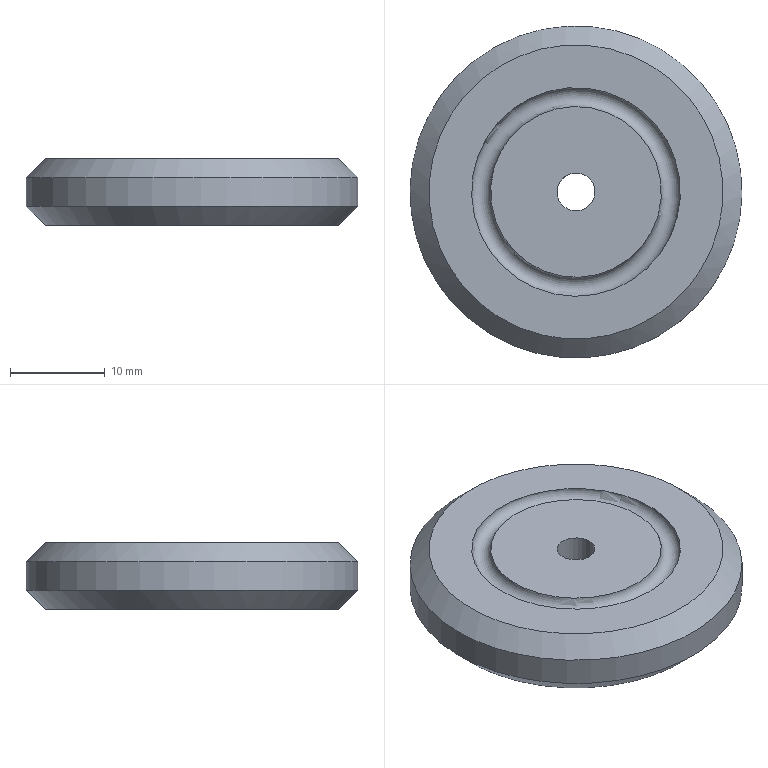Component | NX | SPRING_SEAT | 1 solid | 9 faces | box 35 x 35 x 7 mm | volume 6040 mm3 | cone 3 | plane 3 | cylinder 2 | torus 1 | commonest cylinder face diameters 4 x1 35 x1
STEP:
#1=CARTESIAN_POINT('',(0.,0.,0.));
#2=DIRECTION('',(0.,0.,1.));
#3=DIRECTION('',(1.,0.,0.));
#4=AXIS2_PLACEMENT_3D('',#1,#2,#3);
#5=CARTESIAN_POINT('',(-147.543,-1.847,125.));
#6=VERTEX_POINT('',#5);
#7=CARTESIAN_POINT('',(-146.777,0.,125.));
#8=DIRECTION('',(0.,0.,-1.));
#9=DIRECTION('',(-0.383,-0.9237,0.));
#10=AXIS2_PLACEMENT_3D('',#7,#8,#9);
#11=CIRCLE('',#10,2.);
#12=CARTESIAN_POINT('',(-146.777,0.,122.));
#13=DIRECTION('',(0.,0.,-1.));
#14=DIRECTION('',(-0.383,-0.9237,0.));
#15=AXIS2_PLACEMENT_3D('',#12,#13,#14);
#16=CYLINDRICAL_SURFACE('',#15,2.);
#17=CARTESIAN_POINT('',(0.,-3.));
#18=DIRECTION('',(1.,0.));
#19=VECTOR('',#18,1.);
#20=LINE('',#17,#19);
#21=(GEOMETRIC_REPRESENTATION_CONTEXT(2)PARAMETRIC_REPRESENTATION_CONTEXT()REPRESENTATION_CONTEXT('',''));
#22=DEFINITIONAL_REPRESENTATION('',(#20),#21);
#23=PCURVE('',#16,#22);
#24=CARTESIAN_POINT('',(-146.777,0.,125.));
#25=DIRECTION('',(0.,0.,-1.));
#26=DIRECTION('',(-0.383,-0.9237,0.));
#27=AXIS2_PLACEMENT_3D('',#24,#25,#26);
#28=CONICAL_SURFACE('',#27,2.,0.7854);
#29=CARTESIAN_POINT('',(0.,0.));
#30=DIRECTION('',(1.,0.));
#31=VECTOR('',#30,1.);
#32=LINE('',#29,#31);
#33=(GEOMETRIC_REPRESENTATION_CONTEXT(2)PARAMETRIC_REPRESENTATION_CONTEXT()REPRESENTATION_CONTEXT('',''));
#34=DEFINITIONAL_REPRESENTATION('',(#32),#33);
#35=PCURVE('',#28,#34);
#36=SURFACE_CURVE('',#11,(#23,#35),.PCURVE_S1.);
#37=EDGE_CURVE('',#6,#6,#36,.T.);
#38=ORIENTED_EDGE('',*,*,#37,.F.);
#39=CARTESIAN_POINT('',(-147.543,-1.847,129.));
#40=VERTEX_POINT('',#39);
#41=CARTESIAN_POINT('',(-147.543,-1.847,129.));
#42=CARTESIAN_POINT('',(-147.543,-1.847,125.));
#43=B_SPLINE_CURVE_WITH_KNOTS('',1,(#41,#42),.UNSPECIFIED.,.F.,.F.,(2,2),(-7.,-3.),.PIECEWISE_BEZIER_KNOTS.);
#44=CARTESIAN_POINT('',(0.,0.));
#45=DIRECTION('',(0.,1.));
#46=VECTOR('',#45,1.);
#47=LINE('',#44,#46);
#48=(GEOMETRIC_REPRESENTATION_CONTEXT(2)PARAMETRIC_REPRESENTATION_CONTEXT()REPRESENTATION_CONTEXT('',''));
#49=DEFINITIONAL_REPRESENTATION('',(#47),#48);
#50=PCURVE('',#16,#49);
#51=CARTESIAN_POINT('',(6.283,0.));
#52=DIRECTION('',(0.,1.));
#53=VECTOR('',#52,1.);
#54=LINE('',#51,#53);
#55=(GEOMETRIC_REPRESENTATION_CONTEXT(2)PARAMETRIC_REPRESENTATION_CONTEXT()REPRESENTATION_CONTEXT('',''));
#56=DEFINITIONAL_REPRESENTATION('',(#54),#55);
#57=PCURVE('',#16,#56);
#58=SEAM_CURVE('',#43,(#50,#57),.PCURVE_S1.);
#59=EDGE_CURVE('',#40,#6,#58,.T.);
#60=ORIENTED_EDGE('',*,*,#59,.F.);
#61=CARTESIAN_POINT('',(-146.777,0.,129.));
#62=DIRECTION('',(0.,0.,-1.));
#63=DIRECTION('',(-0.383,-0.9237,0.));
#64=AXIS2_PLACEMENT_3D('',#61,#62,#63);
#65=CIRCLE('',#64,2.);
#66=CARTESIAN_POINT('',(0.,-7.));
#67=DIRECTION('',(1.,0.));
#68=VECTOR('',#67,1.);
#69=LINE('',#66,#68);
#70=(GEOMETRIC_REPRESENTATION_CONTEXT(2)PARAMETRIC_REPRESENTATION_CONTEXT()REPRESENTATION_CONTEXT('',''));
#71=DEFINITIONAL_REPRESENTATION('',(#69),#70);
#72=PCURVE('',#16,#71);
#73=CARTESIAN_POINT('',(-155.091,3.447,129.));
#74=DIRECTION('',(0.,0.,1.));
#75=DIRECTION('',(0.383,0.9237,0.));
#76=AXIS2_PLACEMENT_3D('',#73,#74,#75);
#77=PLANE('',#76);
#78=CARTESIAN_POINT('',(-2.,-9.));
#79=CARTESIAN_POINT('',(-2.,-5.536));
#80=CARTESIAN_POINT('',(1.,-7.268));
#81=CARTESIAN_POINT('',(4.,-9.));
#82=CARTESIAN_POINT('',(1.,-10.732));
#83=CARTESIAN_POINT('',(-2.,-12.464));
#84=CARTESIAN_POINT('',(-2.,-9.));
#85=(BOUNDED_CURVE()B_SPLINE_CURVE(2,(#78,#79,#80,#81,#82,#83,#84),.UNSPECIFIED.,.T.,.F.)B_SPLINE_CURVE_WITH_KNOTS((1,2,2,2,2,1),(-2.094,0.,2.094,4.189,6.283,8.378),.UNSPECIFIED.)CURVE()GEOMETRIC_REPRESENTATION_ITEM()RATIONAL_B_SPLINE_CURVE((1.,0.5,1.,0.5,1.,0.5,1.))REPRESENTATION_ITEM(''));
#86=(GEOMETRIC_REPRESENTATION_CONTEXT(2)PARAMETRIC_REPRESENTATION_CONTEXT()REPRESENTATION_CONTEXT('',''));
#87=DEFINITIONAL_REPRESENTATION('',(#85),#86);
#88=PCURVE('',#77,#87);
#89=SURFACE_CURVE('',#65,(#72,#88),.PCURVE_S1.);
#90=EDGE_CURVE('',#40,#40,#89,.T.);
#91=ORIENTED_EDGE('',*,*,#90,.T.);
#92=ORIENTED_EDGE('',*,*,#59,.T.);
#93=EDGE_LOOP('',(#38,#60,#91,#92));
#94=FACE_BOUND('',#93,.F.);
#95=ADVANCED_FACE('',(#94),#16,.F.);
#96=CARTESIAN_POINT('',(-148.693,-4.619,122.));
#97=VERTEX_POINT('',#96);
#98=CARTESIAN_POINT('',(-146.777,0.,122.));
#99=DIRECTION('',(0.,0.,-1.));
#100=DIRECTION('',(-0.383,-0.9237,0.));
#101=AXIS2_PLACEMENT_3D('',#98,#99,#100);
#102=CIRCLE('',#101,5.);
#103=CARTESIAN_POINT('',(0.,3.));
#104=DIRECTION('',(1.,0.));
#105=VECTOR('',#104,1.);
#106=LINE('',#103,#105);
#107=(GEOMETRIC_REPRESENTATION_CONTEXT(2)PARAMETRIC_REPRESENTATION_CONTEXT()REPRESENTATION_CONTEXT('',''));
#108=DEFINITIONAL_REPRESENTATION('',(#106),#107);
#109=PCURVE('',#28,#108);
#110=CARTESIAN_POINT('',(-151.396,1.915,122.));
#111=DIRECTION('',(0.,0.,-1.));
#112=DIRECTION('',(-0.383,-0.9237,0.));
#113=AXIS2_PLACEMENT_3D('',#110,#111,#112);
#114=PLANE('',#113);
#115=CARTESIAN_POINT('',(-0.,-5.));
#116=DIRECTION('',(1.,-0.));
#117=AXIS2_PLACEMENT_2D('',#115,#116);
#118=CIRCLE('',#117,5.);
#119=(GEOMETRIC_REPRESENTATION_CONTEXT(2)PARAMETRIC_REPRESENTATION_CONTEXT()REPRESENTATION_CONTEXT('',''));
#120=DEFINITIONAL_REPRESENTATION('',(#118),#119);
#121=PCURVE('',#114,#120);
#122=SURFACE_CURVE('',#102,(#109,#121),.PCURVE_S1.);
#123=EDGE_CURVE('',#97,#97,#122,.T.);
#124=ORIENTED_EDGE('',*,*,#123,.F.);
#125=CARTESIAN_POINT('',(-147.543,-1.847,125.));
#126=CARTESIAN_POINT('',(-148.693,-4.619,122.));
#127=B_SPLINE_CURVE_WITH_KNOTS('',1,(#125,#126),.UNSPECIFIED.,.F.,.F.,(2,2),(0.,4.243),.PIECEWISE_BEZIER_KNOTS.);
#128=CARTESIAN_POINT('',(0.,0.));
#129=DIRECTION('',(0.,1.));
#130=VECTOR('',#129,1.);
#131=LINE('',#128,#130);
#132=(GEOMETRIC_REPRESENTATION_CONTEXT(2)PARAMETRIC_REPRESENTATION_CONTEXT()REPRESENTATION_CONTEXT('',''));
#133=DEFINITIONAL_REPRESENTATION('',(#131),#132);
#134=PCURVE('',#28,#133);
#135=CARTESIAN_POINT('',(6.283,0.));
#136=DIRECTION('',(0.,1.));
#137=VECTOR('',#136,1.);
#138=LINE('',#135,#137);
#139=(GEOMETRIC_REPRESENTATION_CONTEXT(2)PARAMETRIC_REPRESENTATION_CONTEXT()REPRESENTATION_CONTEXT('',''));
#140=DEFINITIONAL_REPRESENTATION('',(#138),#139);
#141=PCURVE('',#28,#140);
#142=SEAM_CURVE('',#127,(#134,#141),.PCURVE_S1.);
#143=EDGE_CURVE('',#6,#97,#142,.T.);
#144=ORIENTED_EDGE('',*,*,#143,.F.);
#145=ORIENTED_EDGE('',*,*,#37,.T.);
#146=ORIENTED_EDGE('',*,*,#143,.T.);
#147=EDGE_LOOP('',(#124,#144,#145,#146));
#148=FACE_BOUND('',#147,.F.);
#149=ADVANCED_FACE('',(#148),#28,.F.);
#150=CARTESIAN_POINT('',(-152.715,-14.318,122.));
#151=VERTEX_POINT('',#150);
#152=CARTESIAN_POINT('',(-146.777,0.,122.));
#153=DIRECTION('',(0.,0.,-1.));
#154=DIRECTION('',(-0.383,-0.9237,0.));
#155=AXIS2_PLACEMENT_3D('',#152,#153,#154);
#156=CIRCLE('',#155,15.5);
#157=CARTESIAN_POINT('',(-0.,-5.));
#158=DIRECTION('',(1.,0.));
#159=AXIS2_PLACEMENT_2D('',#157,#158);
#160=CIRCLE('',#159,15.5);
#161=(GEOMETRIC_REPRESENTATION_CONTEXT(2)PARAMETRIC_REPRESENTATION_CONTEXT()REPRESENTATION_CONTEXT('',''));
#162=DEFINITIONAL_REPRESENTATION('',(#160),#161);
#163=PCURVE('',#114,#162);
#164=CARTESIAN_POINT('',(-146.777,0.,122.));
#165=DIRECTION('',(0.,0.,1.));
#166=DIRECTION('',(0.383,0.9237,0.));
#167=AXIS2_PLACEMENT_3D('',#164,#165,#166);
#168=CONICAL_SURFACE('',#167,15.5,0.7854);
#169=CARTESIAN_POINT('',(9.425,0.));
#170=DIRECTION('',(-1.,0.));
#171=VECTOR('',#170,1.);
#172=LINE('',#169,#171);
#173=(GEOMETRIC_REPRESENTATION_CONTEXT(2)PARAMETRIC_REPRESENTATION_CONTEXT()REPRESENTATION_CONTEXT('',''));
#174=DEFINITIONAL_REPRESENTATION('',(#172),#173);
#175=PCURVE('',#168,#174);
#176=SURFACE_CURVE('',#156,(#163,#175),.PCURVE_S1.);
#177=EDGE_CURVE('',#151,#151,#176,.T.);
#178=ORIENTED_EDGE('',*,*,#177,.T.);
#179=EDGE_LOOP('',(#178));
#180=FACE_BOUND('',#179,.T.);
#181=ORIENTED_EDGE('',*,*,#123,.F.);
#182=EDGE_LOOP('',(#181));
#183=FACE_BOUND('',#182,.T.);
#184=ADVANCED_FACE('',(#180,#183),#114,.T.);
#185=CARTESIAN_POINT('',(-153.481,-16.165,124.));
#186=VERTEX_POINT('',#185);
#187=CARTESIAN_POINT('',(-146.777,0.,124.));
#188=DIRECTION('',(0.,0.,-1.));
#189=DIRECTION('',(-0.383,-0.9237,0.));
#190=AXIS2_PLACEMENT_3D('',#187,#188,#189);
#191=CIRCLE('',#190,17.5);
#192=CARTESIAN_POINT('',(9.425,2.));
#193=DIRECTION('',(-1.,0.));
#194=VECTOR('',#193,1.);
#195=LINE('',#192,#194);
#196=(GEOMETRIC_REPRESENTATION_CONTEXT(2)PARAMETRIC_REPRESENTATION_CONTEXT()REPRESENTATION_CONTEXT('',''));
#197=DEFINITIONAL_REPRESENTATION('',(#195),#196);
#198=PCURVE('',#168,#197);
#199=CARTESIAN_POINT('',(-146.777,0.,122.));
#200=DIRECTION('',(0.,0.,-1.));
#201=DIRECTION('',(-0.383,-0.9237,0.));
#202=AXIS2_PLACEMENT_3D('',#199,#200,#201);
#203=CYLINDRICAL_SURFACE('',#202,17.5);
#204=CARTESIAN_POINT('',(0.,-2.));
#205=DIRECTION('',(1.,0.));
#206=VECTOR('',#205,1.);
#207=LINE('',#204,#206);
#208=(GEOMETRIC_REPRESENTATION_CONTEXT(2)PARAMETRIC_REPRESENTATION_CONTEXT()REPRESENTATION_CONTEXT('',''));
#209=DEFINITIONAL_REPRESENTATION('',(#207),#208);
#210=PCURVE('',#203,#209);
#211=SURFACE_CURVE('',#191,(#198,#210),.PCURVE_S1.);
#212=EDGE_CURVE('',#186,#186,#211,.T.);
#213=ORIENTED_EDGE('',*,*,#212,.T.);
#214=CARTESIAN_POINT('',(-152.715,-14.318,122.));
#215=CARTESIAN_POINT('',(-153.481,-16.165,124.));
#216=B_SPLINE_CURVE_WITH_KNOTS('',1,(#214,#215),.UNSPECIFIED.,.F.,.F.,(2,2),(0.,2.828),.PIECEWISE_BEZIER_KNOTS.);
#217=CARTESIAN_POINT('',(3.142,0.));
#218=DIRECTION('',(0.,1.));
#219=VECTOR('',#218,1.);
#220=LINE('',#217,#219);
#221=(GEOMETRIC_REPRESENTATION_CONTEXT(2)PARAMETRIC_REPRESENTATION_CONTEXT()REPRESENTATION_CONTEXT('',''));
#222=DEFINITIONAL_REPRESENTATION('',(#220),#221);
#223=PCURVE('',#168,#222);
#224=CARTESIAN_POINT('',(9.425,0.));
#225=DIRECTION('',(0.,1.));
#226=VECTOR('',#225,1.);
#227=LINE('',#224,#226);
#228=(GEOMETRIC_REPRESENTATION_CONTEXT(2)PARAMETRIC_REPRESENTATION_CONTEXT()REPRESENTATION_CONTEXT('',''));
#229=DEFINITIONAL_REPRESENTATION('',(#227),#228);
#230=PCURVE('',#168,#229);
#231=SEAM_CURVE('',#216,(#223,#230),.PCURVE_S1.);
#232=EDGE_CURVE('',#151,#186,#231,.T.);
#233=ORIENTED_EDGE('',*,*,#232,.F.);
#234=ORIENTED_EDGE('',*,*,#177,.F.);
#235=ORIENTED_EDGE('',*,*,#232,.T.);
#236=EDGE_LOOP('',(#213,#233,#234,#235));
#237=FACE_BOUND('',#236,.T.);
#238=ADVANCED_FACE('',(#237),#168,.T.);
#239=CARTESIAN_POINT('',(-153.481,-16.165,127.));
#240=VERTEX_POINT('',#239);
#241=CARTESIAN_POINT('',(-146.777,0.,127.));
#242=DIRECTION('',(0.,0.,-1.));
#243=DIRECTION('',(-0.383,-0.9237,0.));
#244=AXIS2_PLACEMENT_3D('',#241,#242,#243);
#245=CIRCLE('',#244,17.5);
#246=CARTESIAN_POINT('',(0.,-5.));
#247=DIRECTION('',(1.,0.));
#248=VECTOR('',#247,1.);
#249=LINE('',#246,#248);
#250=(GEOMETRIC_REPRESENTATION_CONTEXT(2)PARAMETRIC_REPRESENTATION_CONTEXT()REPRESENTATION_CONTEXT('',''));
#251=DEFINITIONAL_REPRESENTATION('',(#249),#250);
#252=PCURVE('',#203,#251);
#253=CARTESIAN_POINT('',(-146.777,0.,127.));
#254=DIRECTION('',(0.,0.,-1.));
#255=DIRECTION('',(-0.383,-0.9237,0.));
#256=AXIS2_PLACEMENT_3D('',#253,#254,#255);
#257=CONICAL_SURFACE('',#256,17.5,0.7854);
#258=CARTESIAN_POINT('',(0.,0.));
#259=DIRECTION('',(1.,0.));
#260=VECTOR('',#259,1.);
#261=LINE('',#258,#260);
#262=(GEOMETRIC_REPRESENTATION_CONTEXT(2)PARAMETRIC_REPRESENTATION_CONTEXT()REPRESENTATION_CONTEXT('',''));
#263=DEFINITIONAL_REPRESENTATION('',(#261),#262);
#264=PCURVE('',#257,#263);
#265=SURFACE_CURVE('',#245,(#252,#264),.PCURVE_S1.);
#266=EDGE_CURVE('',#240,#240,#265,.T.);
#267=ORIENTED_EDGE('',*,*,#266,.T.);
#268=CARTESIAN_POINT('',(-153.481,-16.165,127.));
#269=CARTESIAN_POINT('',(-153.481,-16.165,124.));
#270=B_SPLINE_CURVE_WITH_KNOTS('',1,(#268,#269),.UNSPECIFIED.,.F.,.F.,(2,2),(-5.,-2.),.PIECEWISE_BEZIER_KNOTS.);
#271=CARTESIAN_POINT('',(6.283,0.));
#272=DIRECTION('',(0.,1.));
#273=VECTOR('',#272,1.);
#274=LINE('',#271,#273);
#275=(GEOMETRIC_REPRESENTATION_CONTEXT(2)PARAMETRIC_REPRESENTATION_CONTEXT()REPRESENTATION_CONTEXT('',''));
#276=DEFINITIONAL_REPRESENTATION('',(#274),#275);
#277=PCURVE('',#203,#276);
#278=CARTESIAN_POINT('',(0.,0.));
#279=DIRECTION('',(0.,1.));
#280=VECTOR('',#279,1.);
#281=LINE('',#278,#280);
#282=(GEOMETRIC_REPRESENTATION_CONTEXT(2)PARAMETRIC_REPRESENTATION_CONTEXT()REPRESENTATION_CONTEXT('',''));
#283=DEFINITIONAL_REPRESENTATION('',(#281),#282);
#284=PCURVE('',#203,#283);
#285=SEAM_CURVE('',#270,(#277,#284),.PCURVE_S1.);
#286=EDGE_CURVE('',#240,#186,#285,.T.);
#287=ORIENTED_EDGE('',*,*,#286,.T.);
#288=ORIENTED_EDGE('',*,*,#212,.F.);
#289=ORIENTED_EDGE('',*,*,#286,.F.);
#290=EDGE_LOOP('',(#267,#287,#288,#289));
#291=FACE_BOUND('',#290,.T.);
#292=ADVANCED_FACE('',(#291),#203,.T.);
#293=CARTESIAN_POINT('',(-152.715,-14.318,129.));
#294=VERTEX_POINT('',#293);
#295=CARTESIAN_POINT('',(-146.777,0.,129.));
#296=DIRECTION('',(0.,0.,-1.));
#297=DIRECTION('',(-0.383,-0.9237,0.));
#298=AXIS2_PLACEMENT_3D('',#295,#296,#297);
#299=CIRCLE('',#298,15.5);
#300=CARTESIAN_POINT('',(0.,-2.));
#301=DIRECTION('',(1.,0.));
#302=VECTOR('',#301,1.);
#303=LINE('',#300,#302);
#304=(GEOMETRIC_REPRESENTATION_CONTEXT(2)PARAMETRIC_REPRESENTATION_CONTEXT()REPRESENTATION_CONTEXT('',''));
#305=DEFINITIONAL_REPRESENTATION('',(#303),#304);
#306=PCURVE('',#257,#305);
#307=CARTESIAN_POINT('',(-161.095,5.937,129.));
#308=DIRECTION('',(0.,0.,1.));
#309=DIRECTION('',(0.383,0.9237,0.));
#310=AXIS2_PLACEMENT_3D('',#307,#308,#309);
#311=PLANE('',#310);
#312=CARTESIAN_POINT('',(-15.5,-15.5));
#313=CARTESIAN_POINT('',(-15.5,11.347));
#314=CARTESIAN_POINT('',(7.75,-2.077));
#315=CARTESIAN_POINT('',(31.,-15.5));
#316=CARTESIAN_POINT('',(7.75,-28.923));
#317=CARTESIAN_POINT('',(-15.5,-42.347));
#318=CARTESIAN_POINT('',(-15.5,-15.5));
#319=(BOUNDED_CURVE()B_SPLINE_CURVE(2,(#312,#313,#314,#315,#316,#317,#318),.UNSPECIFIED.,.T.,.F.)B_SPLINE_CURVE_WITH_KNOTS((1,2,2,2,2,1),(-2.094,0.,2.094,4.189,6.283,8.378),.UNSPECIFIED.)CURVE()GEOMETRIC_REPRESENTATION_ITEM()RATIONAL_B_SPLINE_CURVE((1.,0.5,1.,0.5,1.,0.5,1.))REPRESENTATION_ITEM(''));
#320=(GEOMETRIC_REPRESENTATION_CONTEXT(2)PARAMETRIC_REPRESENTATION_CONTEXT()REPRESENTATION_CONTEXT('',''));
#321=DEFINITIONAL_REPRESENTATION('',(#319),#320);
#322=PCURVE('',#311,#321);
#323=SURFACE_CURVE('',#299,(#306,#322),.PCURVE_S1.);
#324=EDGE_CURVE('',#294,#294,#323,.T.);
#325=ORIENTED_EDGE('',*,*,#324,.T.);
#326=CARTESIAN_POINT('',(-152.715,-14.318,129.));
#327=CARTESIAN_POINT('',(-153.481,-16.165,127.));
#328=B_SPLINE_CURVE_WITH_KNOTS('',1,(#326,#327),.UNSPECIFIED.,.F.,.F.,(2,2),(-2.828,0.),.PIECEWISE_BEZIER_KNOTS.);
#329=CARTESIAN_POINT('',(6.283,0.));
#330=DIRECTION('',(0.,1.));
#331=VECTOR('',#330,1.);
#332=LINE('',#329,#331);
#333=(GEOMETRIC_REPRESENTATION_CONTEXT(2)PARAMETRIC_REPRESENTATION_CONTEXT()REPRESENTATION_CONTEXT('',''));
#334=DEFINITIONAL_REPRESENTATION('',(#332),#333);
#335=PCURVE('',#257,#334);
#336=CARTESIAN_POINT('',(0.,0.));
#337=DIRECTION('',(0.,1.));
#338=VECTOR('',#337,1.);
#339=LINE('',#336,#338);
#340=(GEOMETRIC_REPRESENTATION_CONTEXT(2)PARAMETRIC_REPRESENTATION_CONTEXT()REPRESENTATION_CONTEXT('',''));
#341=DEFINITIONAL_REPRESENTATION('',(#339),#340);
#342=PCURVE('',#257,#341);
#343=SEAM_CURVE('',#328,(#335,#342),.PCURVE_S1.);
#344=EDGE_CURVE('',#294,#240,#343,.T.);
#345=ORIENTED_EDGE('',*,*,#344,.T.);
#346=ORIENTED_EDGE('',*,*,#266,.F.);
#347=ORIENTED_EDGE('',*,*,#344,.F.);
#348=EDGE_LOOP('',(#325,#345,#346,#347));
#349=FACE_BOUND('',#348,.T.);
#350=ADVANCED_FACE('',(#349),#257,.T.);
#351=CARTESIAN_POINT('',(-150.991,-10.161,129.));
#352=VERTEX_POINT('',#351);
#353=CARTESIAN_POINT('',(-146.777,0.,129.));
#354=DIRECTION('',(0.,0.,-1.));
#355=DIRECTION('',(-0.383,-0.9237,0.));
#356=AXIS2_PLACEMENT_3D('',#353,#354,#355);
#357=CIRCLE('',#356,11.);
#358=CARTESIAN_POINT('',(-11.,-15.5));
#359=CARTESIAN_POINT('',(-11.,3.553));
#360=CARTESIAN_POINT('',(5.5,-5.974));
#361=CARTESIAN_POINT('',(22.,-15.5));
#362=CARTESIAN_POINT('',(5.5,-25.026));
#363=CARTESIAN_POINT('',(-11.,-34.553));
#364=CARTESIAN_POINT('',(-11.,-15.5));
#365=(BOUNDED_CURVE()B_SPLINE_CURVE(2,(#358,#359,#360,#361,#362,#363,#364),.UNSPECIFIED.,.T.,.F.)B_SPLINE_CURVE_WITH_KNOTS((1,2,2,2,2,1),(-2.094,0.,2.094,4.189,6.283,8.378),.UNSPECIFIED.)CURVE()GEOMETRIC_REPRESENTATION_ITEM()RATIONAL_B_SPLINE_CURVE((1.,0.5,1.,0.5,1.,0.5,1.))REPRESENTATION_ITEM(''));
#366=(GEOMETRIC_REPRESENTATION_CONTEXT(2)PARAMETRIC_REPRESENTATION_CONTEXT()REPRESENTATION_CONTEXT('',''));
#367=DEFINITIONAL_REPRESENTATION('',(#365),#366);
#368=PCURVE('',#311,#367);
#369=CARTESIAN_POINT('',(-146.777,0.,129.));
#370=DIRECTION('',(0.,0.,-1.));
#371=DIRECTION('',(-0.383,-0.9237,0.));
#372=AXIS2_PLACEMENT_3D('',#369,#370,#371);
#373=TOROIDAL_SURFACE('',#372,10.,1.);
#374=CARTESIAN_POINT('',(0.,6.283));
#375=DIRECTION('',(1.,0.));
#376=VECTOR('',#375,1.);
#377=LINE('',#374,#376);
#378=(GEOMETRIC_REPRESENTATION_CONTEXT(2)PARAMETRIC_REPRESENTATION_CONTEXT()REPRESENTATION_CONTEXT('',''));
#379=DEFINITIONAL_REPRESENTATION('',(#377),#378);
#380=PCURVE('',#373,#379);
#381=SURFACE_CURVE('',#357,(#368,#380),.PCURVE_S1.);
#382=EDGE_CURVE('',#352,#352,#381,.T.);
#383=ORIENTED_EDGE('',*,*,#382,.T.);
#384=EDGE_LOOP('',(#383));
#385=FACE_BOUND('',#384,.T.);
#386=ORIENTED_EDGE('',*,*,#324,.F.);
#387=EDGE_LOOP('',(#386));
#388=FACE_BOUND('',#387,.T.);
#389=ADVANCED_FACE('',(#385,#388),#311,.T.);
#390=CARTESIAN_POINT('',(-150.225,-8.314,129.));
#391=VERTEX_POINT('',#390);
#392=CARTESIAN_POINT('',(-146.777,0.,129.));
#393=DIRECTION('',(0.,0.,-1.));
#394=DIRECTION('',(-0.383,-0.9237,0.));
#395=AXIS2_PLACEMENT_3D('',#392,#393,#394);
#396=CIRCLE('',#395,9.);
#397=CARTESIAN_POINT('',(0.,9.425));
#398=DIRECTION('',(1.,0.));
#399=VECTOR('',#398,1.);
#400=LINE('',#397,#399);
#401=(GEOMETRIC_REPRESENTATION_CONTEXT(2)PARAMETRIC_REPRESENTATION_CONTEXT()REPRESENTATION_CONTEXT('',''));
#402=DEFINITIONAL_REPRESENTATION('',(#400),#401);
#403=PCURVE('',#373,#402);
#404=CARTESIAN_POINT('',(-9.,-9.));
#405=CARTESIAN_POINT('',(-9.,6.588));
#406=CARTESIAN_POINT('',(4.5,-1.206));
#407=CARTESIAN_POINT('',(18.,-9.));
#408=CARTESIAN_POINT('',(4.5,-16.794));
#409=CARTESIAN_POINT('',(-9.,-24.588));
#410=CARTESIAN_POINT('',(-9.,-9.));
#411=(BOUNDED_CURVE()B_SPLINE_CURVE(2,(#404,#405,#406,#407,#408,#409,#410),.UNSPECIFIED.,.T.,.F.)B_SPLINE_CURVE_WITH_KNOTS((1,2,2,2,2,1),(-2.094,0.,2.094,4.189,6.283,8.378),.UNSPECIFIED.)CURVE()GEOMETRIC_REPRESENTATION_ITEM()RATIONAL_B_SPLINE_CURVE((1.,0.5,1.,0.5,1.,0.5,1.))REPRESENTATION_ITEM(''));
#412=(GEOMETRIC_REPRESENTATION_CONTEXT(2)PARAMETRIC_REPRESENTATION_CONTEXT()REPRESENTATION_CONTEXT('',''));
#413=DEFINITIONAL_REPRESENTATION('',(#411),#412);
#414=PCURVE('',#77,#413);
#415=SURFACE_CURVE('',#396,(#403,#414),.PCURVE_S1.);
#416=EDGE_CURVE('',#391,#391,#415,.T.);
#417=ORIENTED_EDGE('',*,*,#416,.F.);
#418=CARTESIAN_POINT('',(-150.991,-10.161,129.));
#419=CARTESIAN_POINT('',(-150.991,-10.161,128.607));
#420=CARTESIAN_POINT('',(-150.923,-9.998,128.215));
#421=CARTESIAN_POINT('',(-150.788,-9.673,127.914));
#422=CARTESIAN_POINT('',(-150.608,-9.237,127.798));
#423=CARTESIAN_POINT('',(-150.427,-8.802,127.914));
#424=CARTESIAN_POINT('',(-150.292,-8.476,128.215));
#425=CARTESIAN_POINT('',(-150.225,-8.314,128.607));
#426=CARTESIAN_POINT('',(-150.225,-8.314,129.));
#427=B_SPLINE_CURVE_WITH_KNOTS('',8,(#418,#419,#420,#421,#422,#423,#424,#425,#426),.UNSPECIFIED.,.F.,.F.,(9,9),(0.,3.142),.PIECEWISE_BEZIER_KNOTS.);
#428=CARTESIAN_POINT('',(0.,6.283));
#429=DIRECTION('',(0.,1.));
#430=VECTOR('',#429,1.);
#431=LINE('',#428,#430);
#432=(GEOMETRIC_REPRESENTATION_CONTEXT(2)PARAMETRIC_REPRESENTATION_CONTEXT()REPRESENTATION_CONTEXT('',''));
#433=DEFINITIONAL_REPRESENTATION('',(#431),#432);
#434=PCURVE('',#373,#433);
#435=CARTESIAN_POINT('',(6.283,6.283));
#436=DIRECTION('',(0.,1.));
#437=VECTOR('',#436,1.);
#438=LINE('',#435,#437);
#439=(GEOMETRIC_REPRESENTATION_CONTEXT(2)PARAMETRIC_REPRESENTATION_CONTEXT()REPRESENTATION_CONTEXT('',''));
#440=DEFINITIONAL_REPRESENTATION('',(#438),#439);
#441=PCURVE('',#373,#440);
#442=SEAM_CURVE('',#427,(#434,#441),.PCURVE_S1.);
#443=EDGE_CURVE('',#352,#391,#442,.T.);
#444=ORIENTED_EDGE('',*,*,#443,.F.);
#445=ORIENTED_EDGE('',*,*,#382,.T.);
#446=ORIENTED_EDGE('',*,*,#443,.T.);
#447=EDGE_LOOP('',(#417,#444,#445,#446));
#448=FACE_BOUND('',#447,.F.);
#449=ADVANCED_FACE('',(#448),#373,.F.);
#450=ORIENTED_EDGE('',*,*,#90,.T.);
#451=EDGE_LOOP('',(#450));
#452=FACE_BOUND('',#451,.T.);
#453=ORIENTED_EDGE('',*,*,#416,.F.);
#454=EDGE_LOOP('',(#453));
#455=FACE_BOUND('',#454,.T.);
#456=ADVANCED_FACE('',(#452,#455),#77,.T.);
#457=CLOSED_SHELL('',(#95,#149,#184,#238,#292,#350,#389,#449,#456));
#458=MANIFOLD_SOLID_BREP('',#457);
#459=(LENGTH_UNIT()NAMED_UNIT(*)SI_UNIT(.MILLI.,.METRE.));
#460=UNCERTAINTY_MEASURE_WITH_UNIT(LENGTH_MEASURE(0.00001),#459,'','');
#461=(NAMED_UNIT(*)PLANE_ANGLE_UNIT()SI_UNIT($,.RADIAN.));
#462=(NAMED_UNIT(*)SI_UNIT($,.STERADIAN.)SOLID_ANGLE_UNIT());
#463=(GEOMETRIC_REPRESENTATION_CONTEXT(3)GLOBAL_UNCERTAINTY_ASSIGNED_CONTEXT((#460))GLOBAL_UNIT_ASSIGNED_CONTEXT((#459,#461,#462))REPRESENTATION_CONTEXT('',''));
#464=ADVANCED_BREP_SHAPE_REPRESENTATION('',(#4,#458),#463);